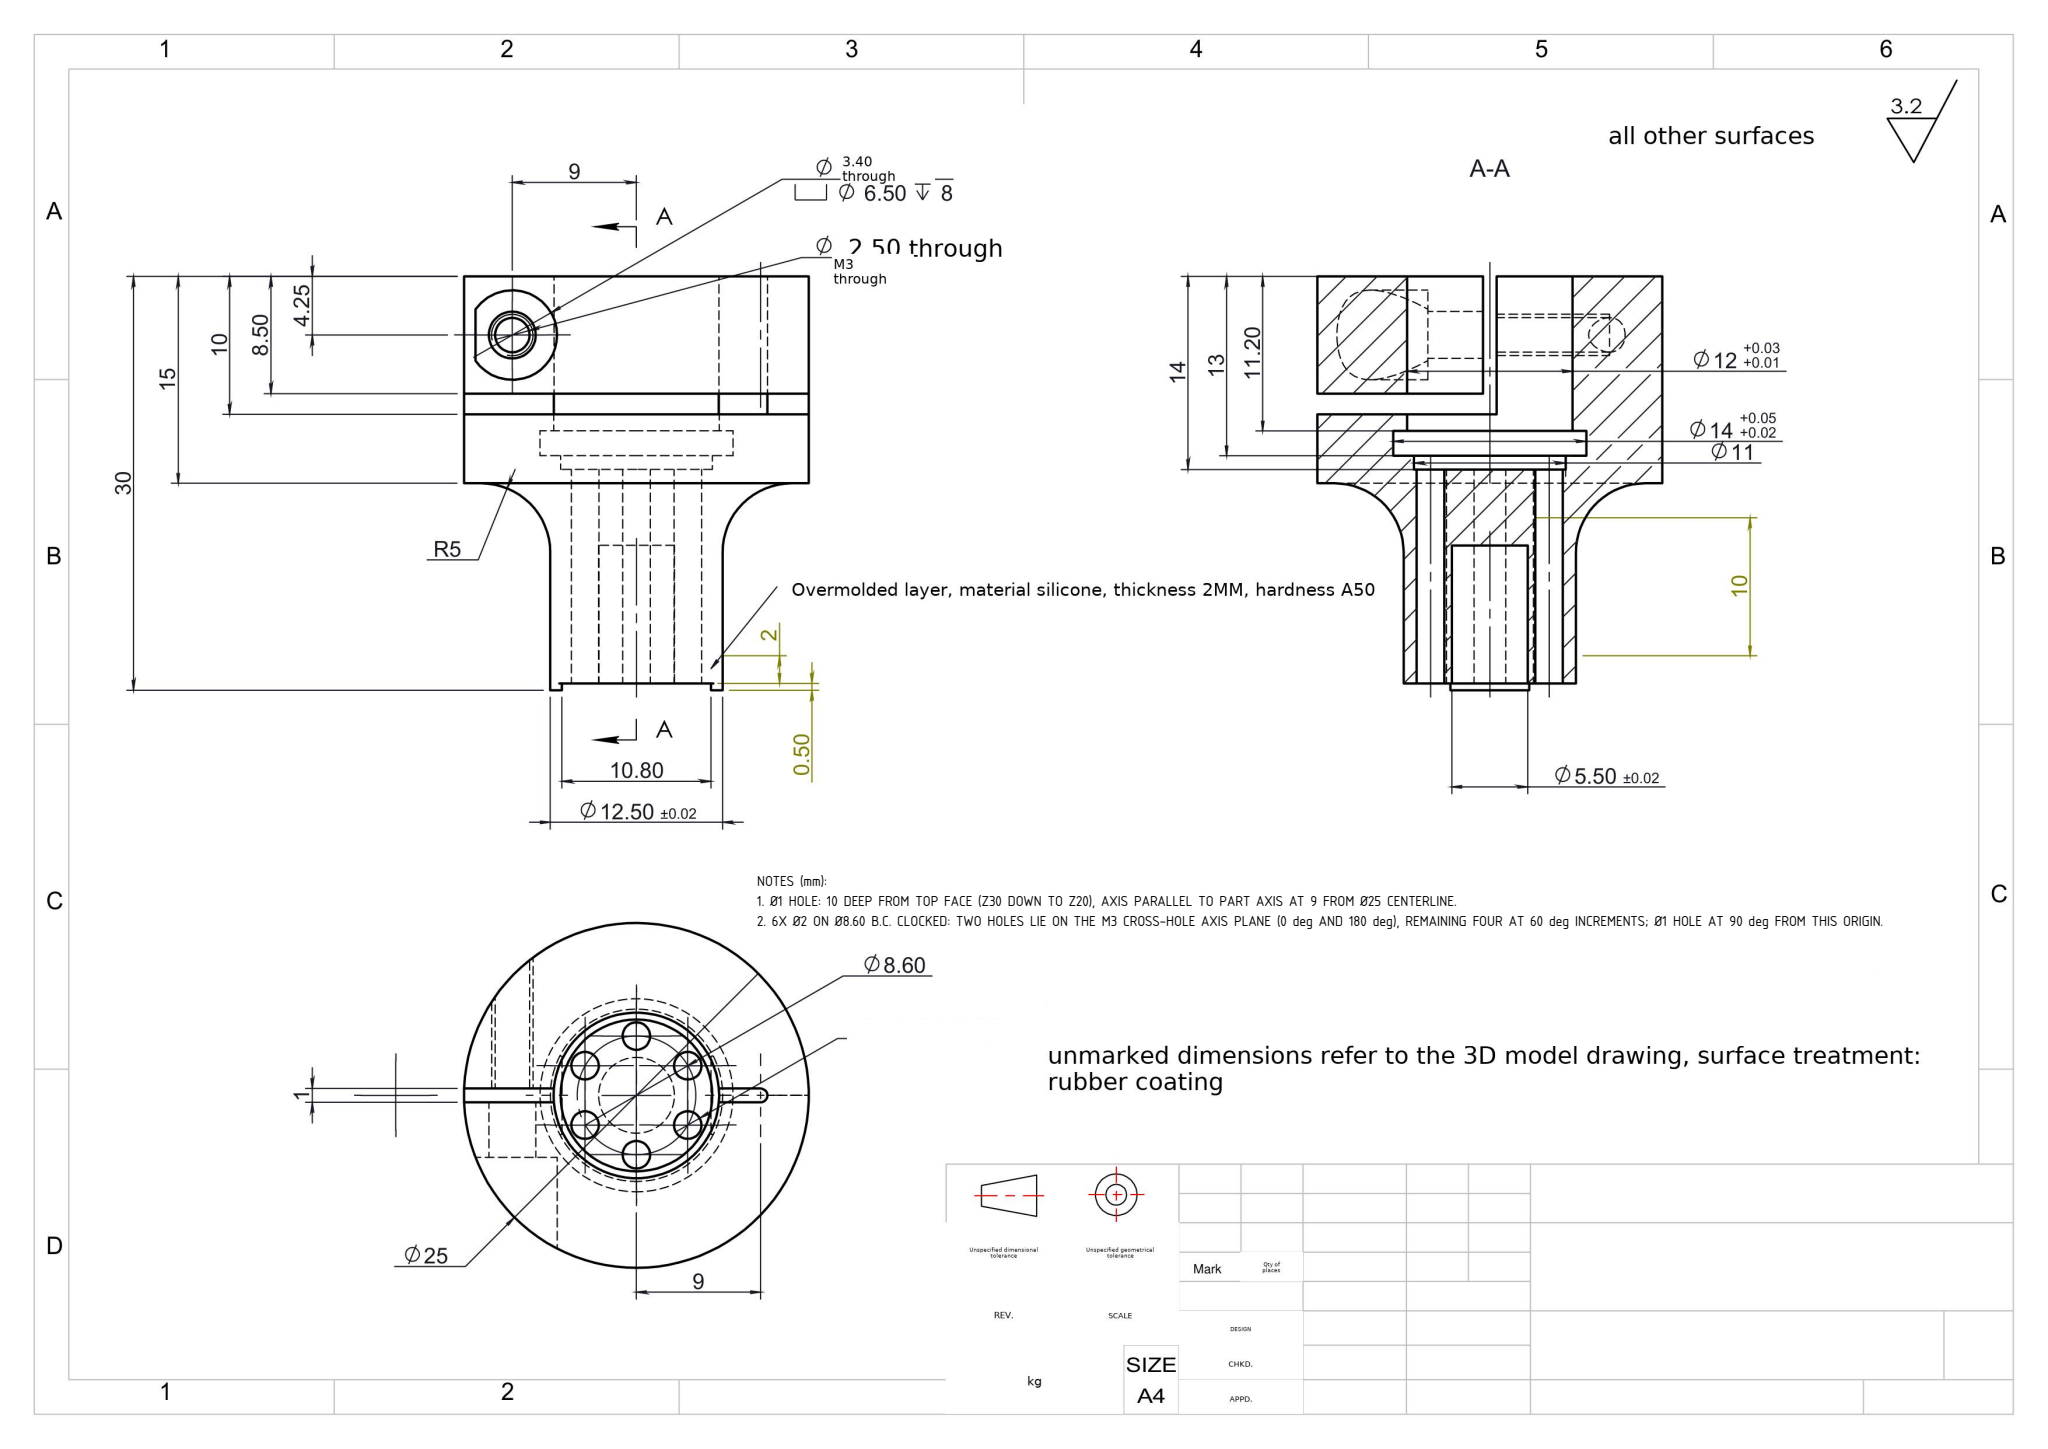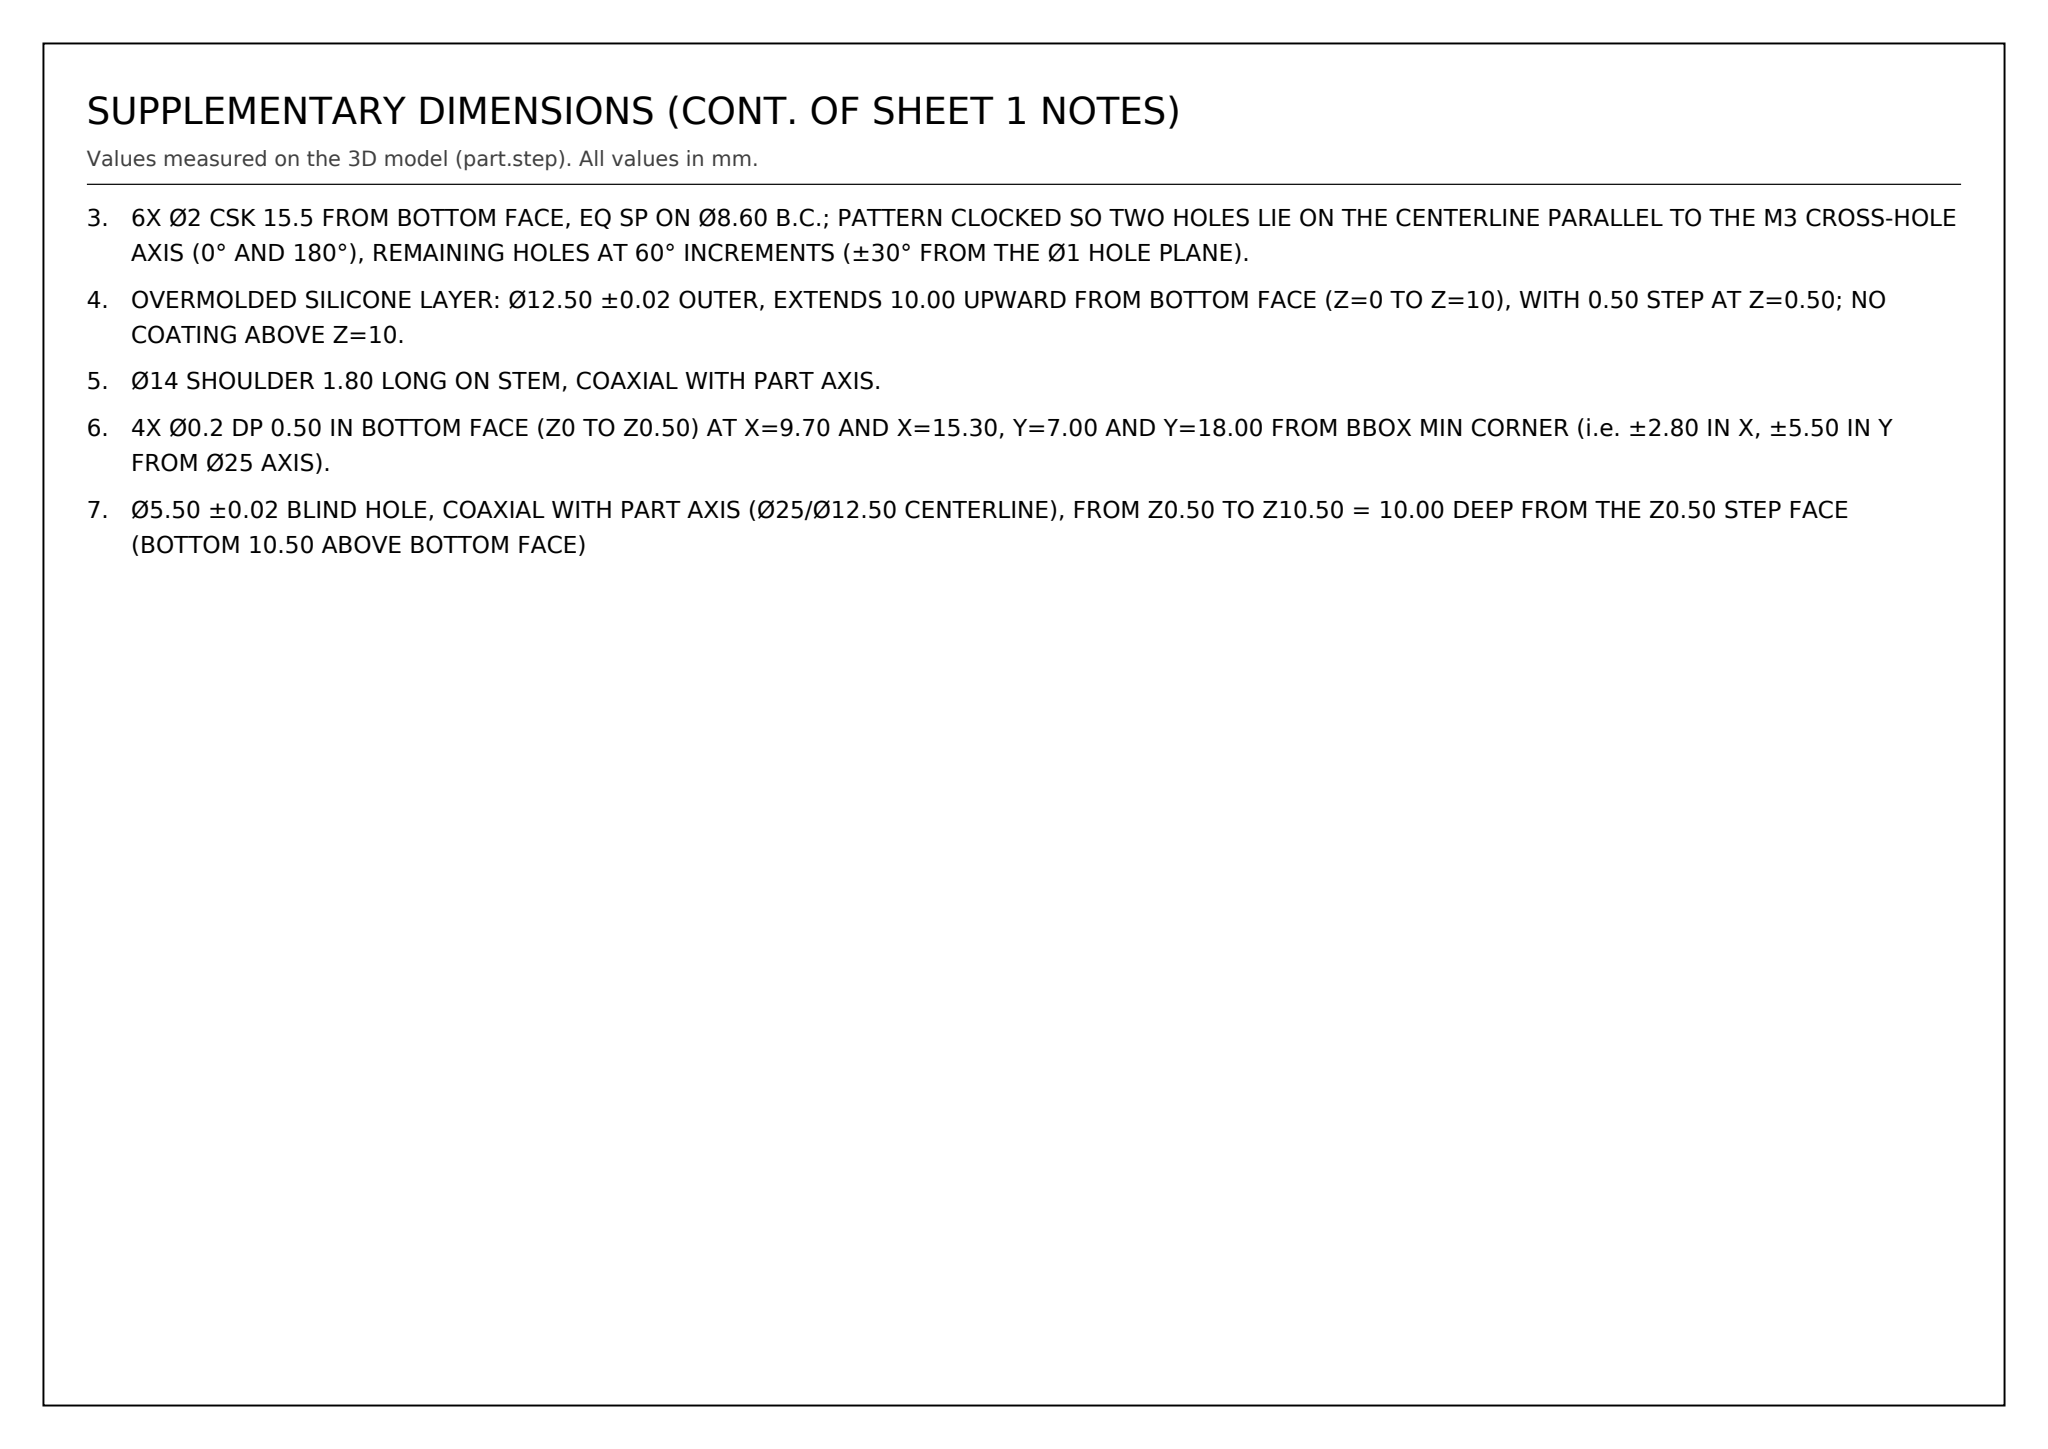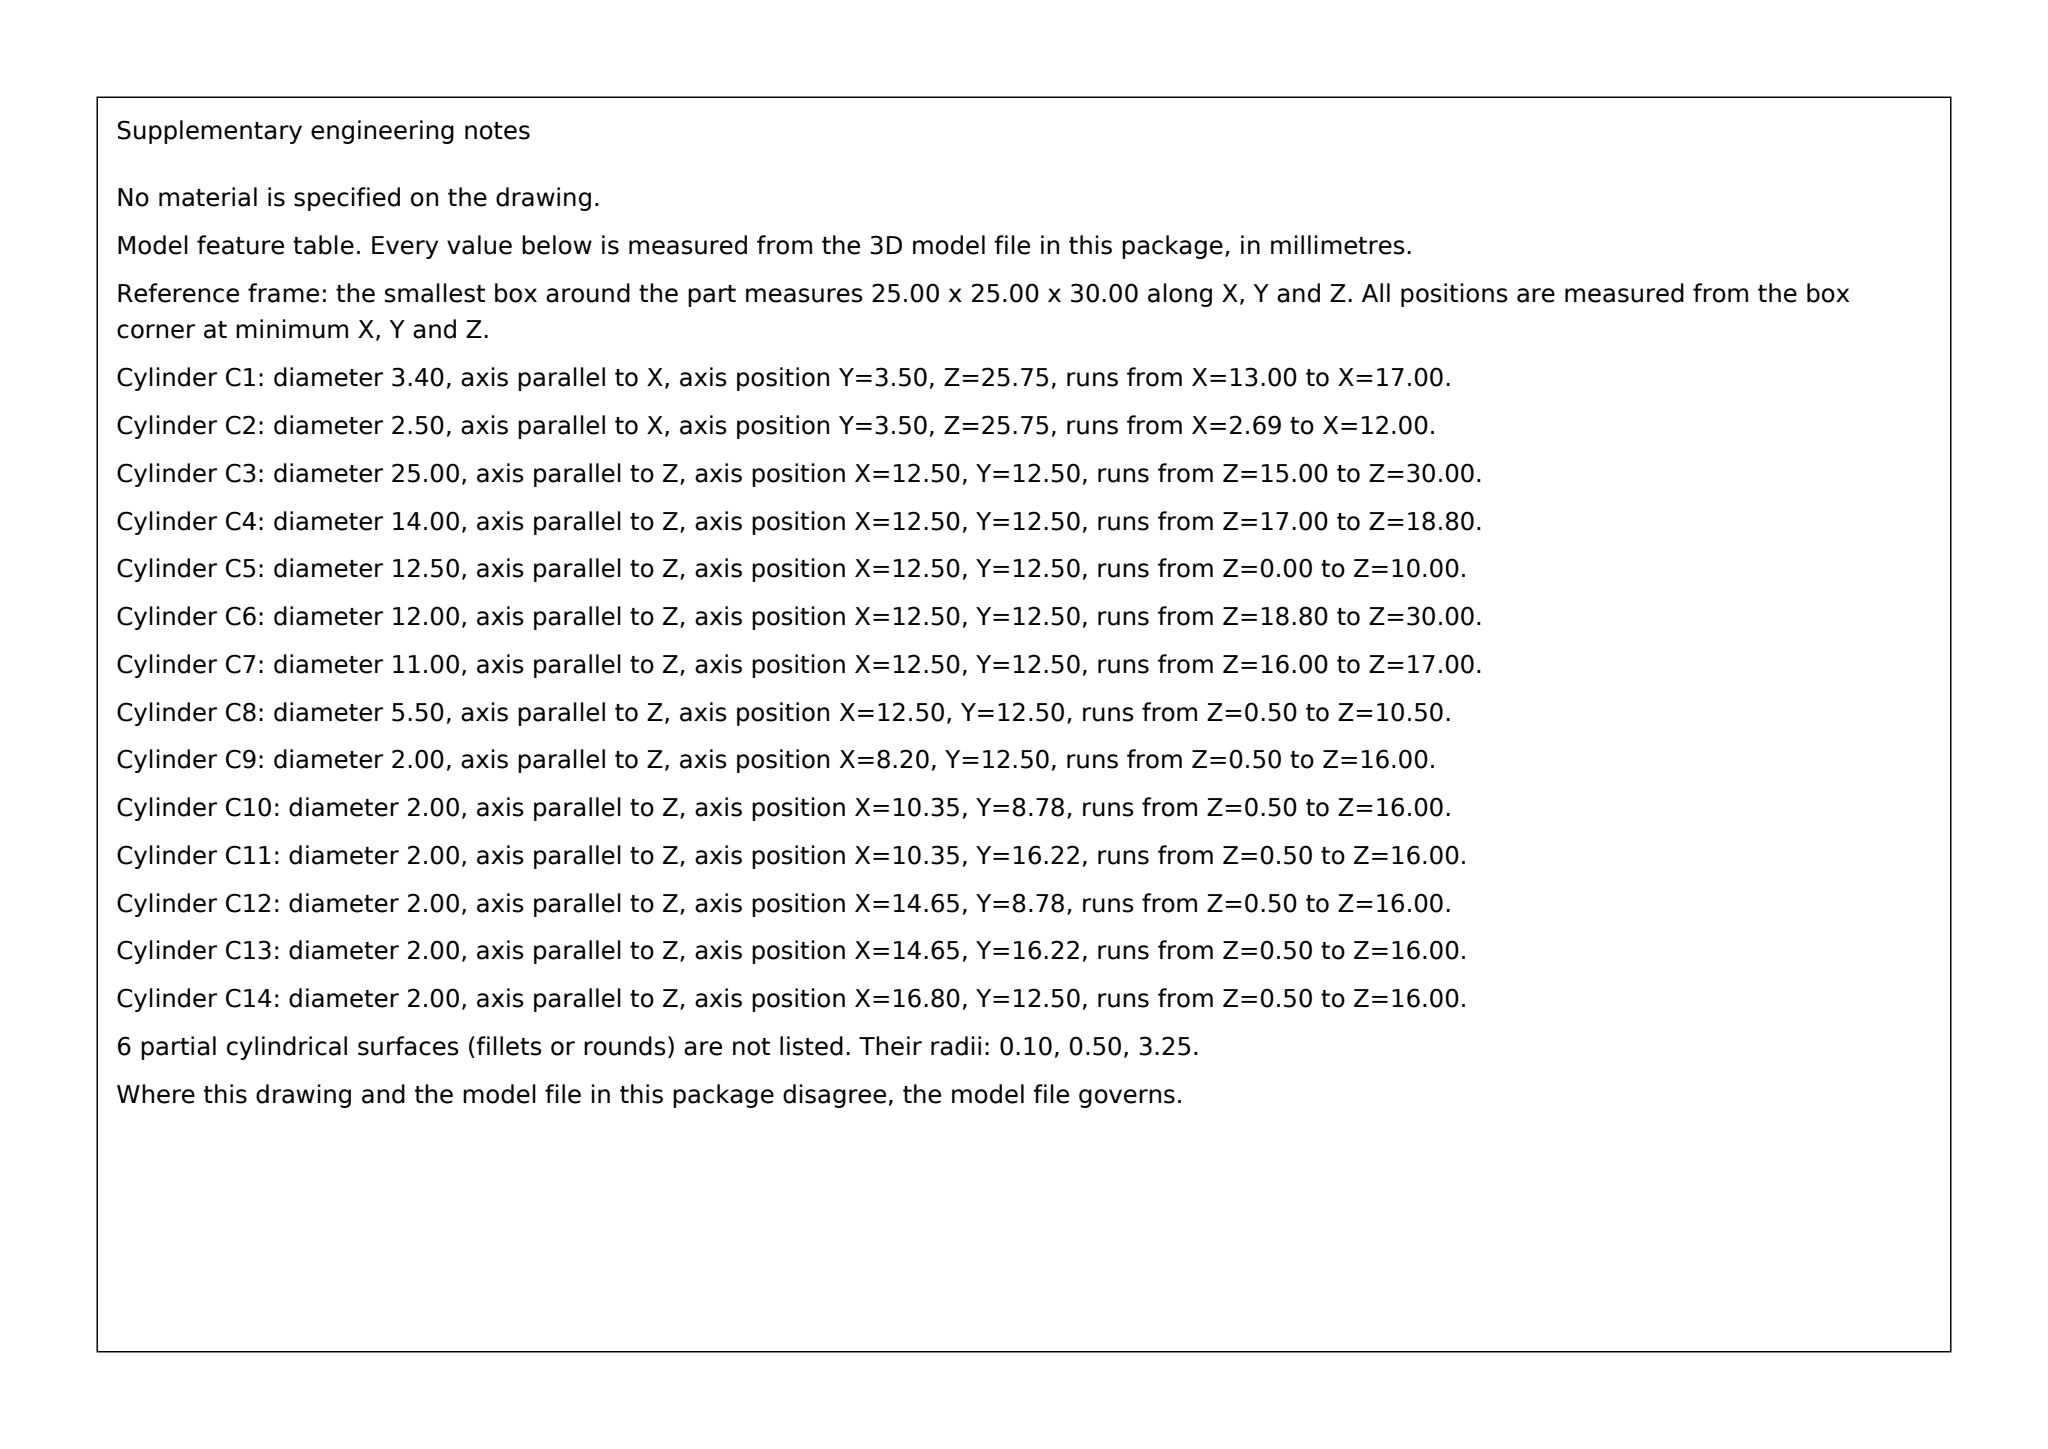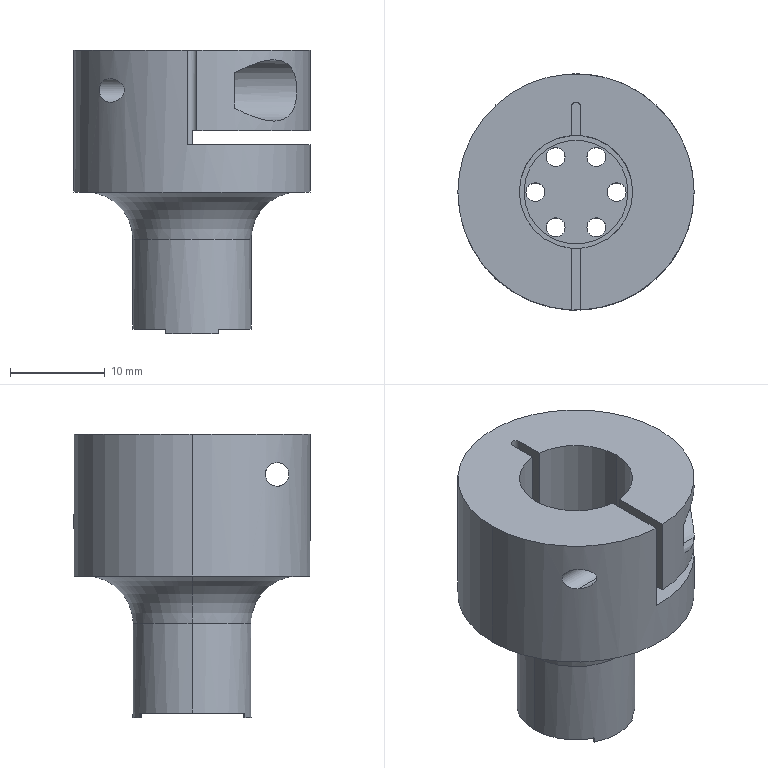Part | SolidWorks | mm | 1 solid | 62 faces | box 25 x 25 x 30 mm | volume 6647 mm3 | cylinder 41 | plane 19 | torus 2 | commonest cylinder face diameters 2 x12 0.2 x6 12 x4 6.5 x3 25 x3 11 x2 2.5 x2 3.4 x2
Drawing notes:
Ø1 HOLE: 10 DEEP FROM TOP FACE (Z30 DOWN TO Z20), AXIS PARALLEL TO PART AXIS AT 9 FROM Ø25 CENTERLINE. | from the solid: cylinder dia 1.0, axis z, pos (12.5, 21.5) = 9 from axis at (12.5,12.5), length 10.0; plane z=20.0
6X Ø2 ON Ø8.60 B.C. CLOCKED: TWO HOLES LIE ON THE M3 CROSS-HOLE AXIS PLANE (0 deg AND 180 deg), REMAINING FOUR AT 60 deg INCREMENTS; Ø1 HOLE AT 90 deg FROM THIS ORIGIN. | from the solid: Ø2 cylinder positions (8.2,12.5),(16.8,12.5),(10.35,8.78),(10.35,16.22),(14.65,8.78),(14.65,16.22) about axis (12.5,12.5) = 0/60/120/180/240/300 deg; M3 axis along x; Ø1 hole at (12.5,21.5) = 90 deg
6X Ø2 CSK 15.5 FROM BOTTOM FACE, EQ SP ON Ø8.60 B.C.; PATTERN CLOCKED SO TWO HOLES LIE ON THE CENTERLINE PARALLEL TO THE M3 CROSS-HOLE AXIS (0° AND 180°), REMAINING HOLES AT 60° INCREMENTS (±30° FROM THE Ø1 HOLE PLANE). | from the solid: 6x cylinders dia 2.0, z axis, length 15.5 at (8.2,12.5),(16.8,12.5),(10.35,8.78),(10.35,16.22),(14.65,8.78),(14.65,16.22) about center (12.5,12.5)
OVERMOLDED SILICONE LAYER: Ø12.50 ±0.02 OUTER, EXTENDS 10.00 UPWARD FROM BOTTOM FACE (Z=0 TO Z=10), WITH 0.50 STEP AT Z=0.50; NO COATING ABOVE Z=10. | from the solid: cylinder [12.5, z, pos (12.5,12.5), length 10]; planes z=0.0, z=0.5, z=10.5
Ø14 SHOULDER 1.80 LONG ON STEM, COAXIAL WITH PART AXIS. | from the solid: cylinder dia 14.0, axis z, pos (12.5,12.5), length 1.8
4X Ø0.2 DP 0.50 IN BOTTOM FACE (Z0 TO Z0.50) AT X=9.70 AND X=15.30, Y=7.00 AND Y=18.00 FROM BBOX MIN CORNER (i.e. ±2.80 IN X, ±5.50 IN Y FROM Ø25 AXIS). | from the solid: Four 0.2 dia arcs with z axis at (9.7,7.0), (9.7,18.0), (15.3,7.0) and (15.3,18.0), each running from z0.0 to z0.5; part axis at X12.5, Y12.5.
Ø5.50 ±0.02 BLIND HOLE, COAXIAL WITH PART AXIS (Ø25/Ø12.50 CENTERLINE), FROM Z0.50 TO Z10.50 = 10.00 DEEP FROM THE Z0.50 STEP FACE (BOTTOM 10.50 ABOVE BOTTOM FACE) | from the solid: cylinders: hole/bore dia 5.5, axis z at [12.5,12.5], from 0.5 to 10.5, 360 deg; axis_plane z=10.5 flat bottom x[9.8,15.3] y[9.8,15.3]